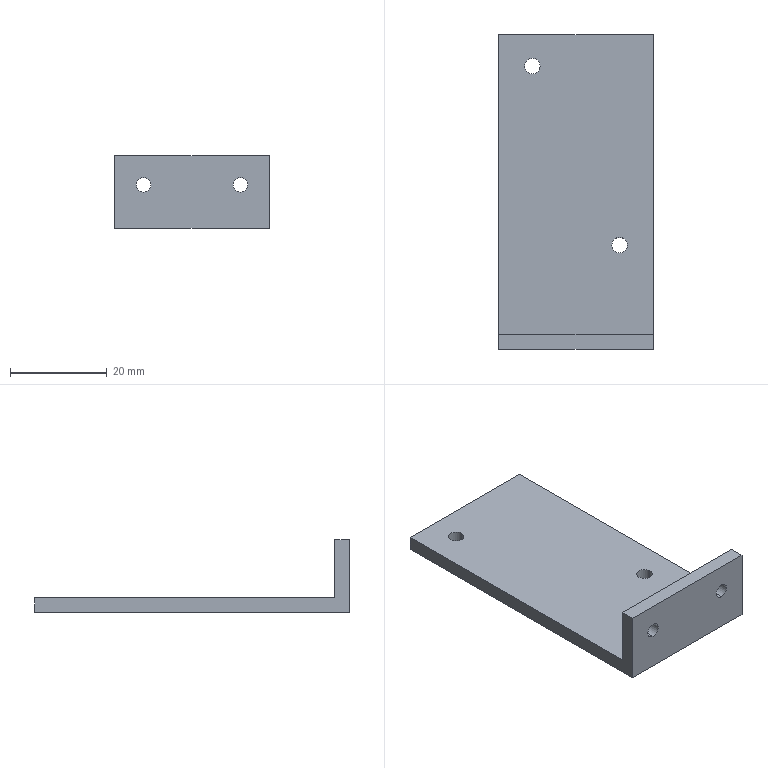CAM job | NX | mm | 3-axis | 3 set-ups | 8 operations | part box 32 x 65 x 15
set-up 1
1. Cavity Milling | Mill Mill5 D8 | CAVITY_MILL | path 3811.381 mm | 13.781 min
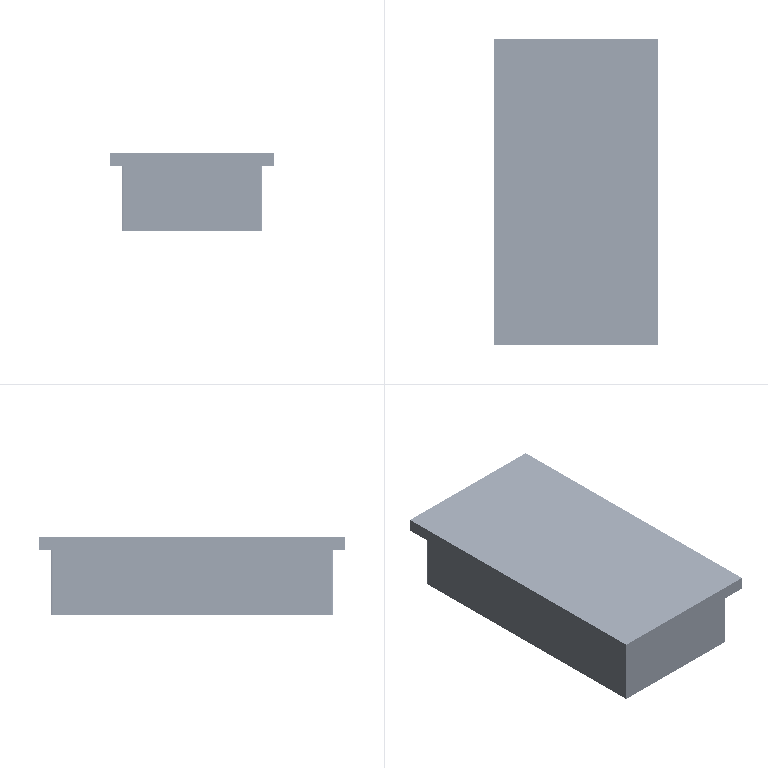2. Cavity Milling | Mill Mill5 D8 | CAVITY_MILL_COPY | path 774.876 mm | 3.022 min
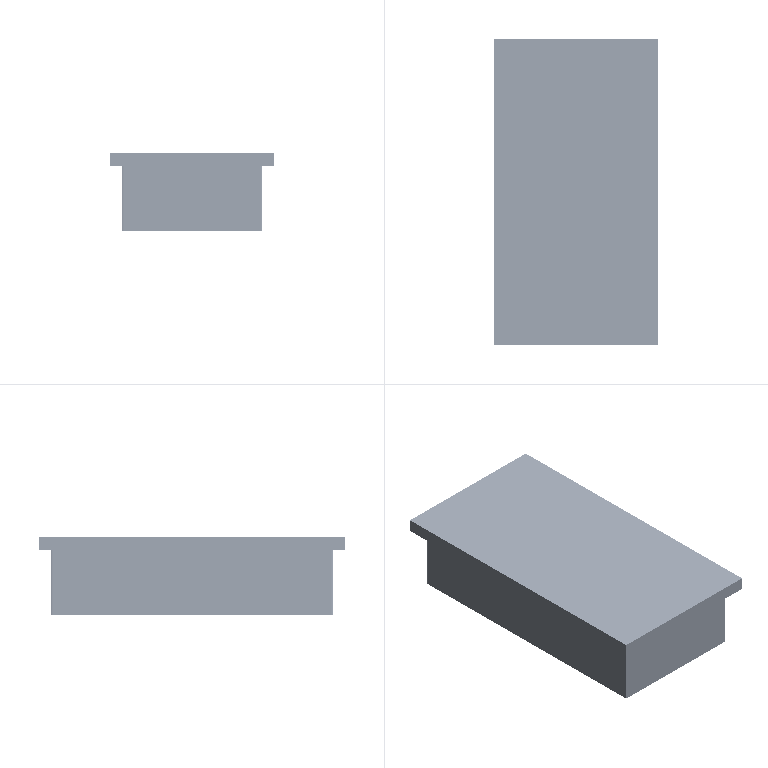3. Planar Milling | Mill Mill5 D8 | PLANAR_PROFILE | path 4093.609 mm | 14.197 min
4. Cylinder Milling | Mill Mill5 D2 | HOLE_MILLING | path 195.726 mm | 0.4196 min
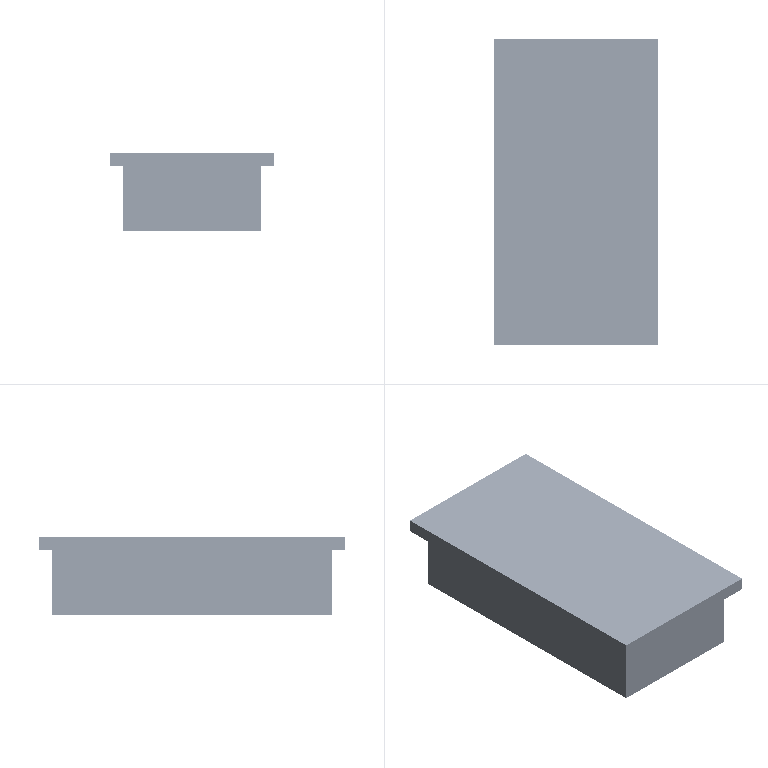set-up 2
5. Cavity Milling | Mill Mill5 D8 | CAVITY_MILL_COPY_1 | path 12025.136 mm | 21.725 min
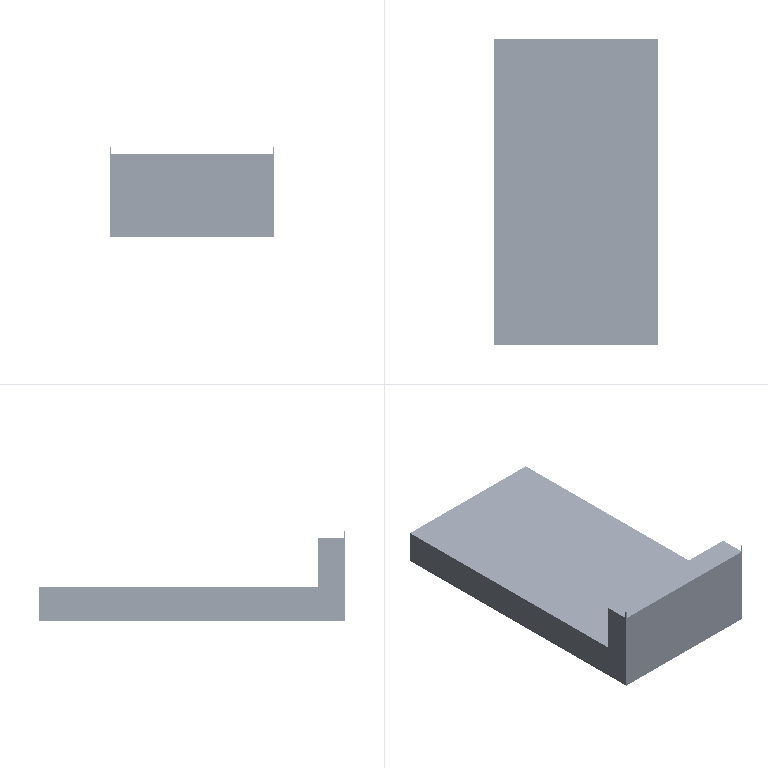6. Volume Based 2.5D Milling | Mill Mill5 D8 | FLOOR_WALL | path 814.765 mm | 2.819 min
7. Planar Milling | Mill Mill5 D8 | PLANAR_PROFILE_COPY | path 948 mm | 2.528 min
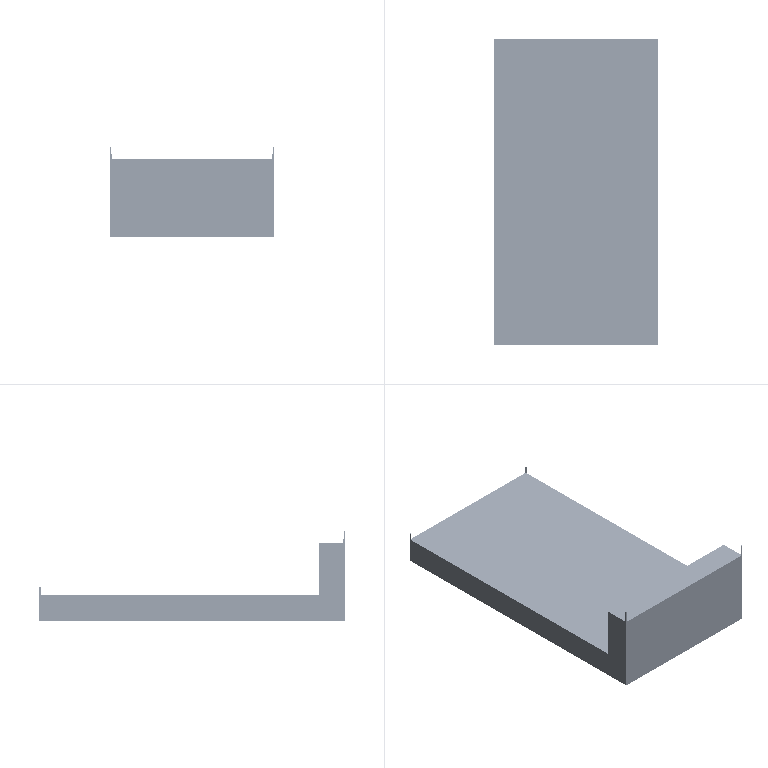set-up 3
8. Cylinder Milling | Mill Mill5 D2 | HOLE_MILLING_COPY | path 157.772 mm | 0.3503 min